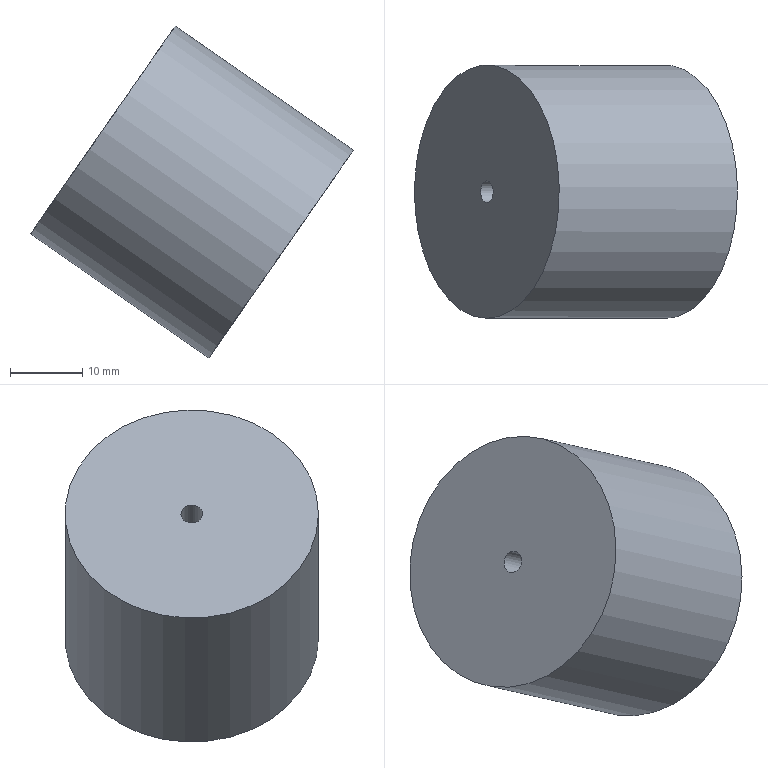Component | NX | SPROCKET_4 | 1 solid | 4 faces | box 44.62 x 35 x 45.87 mm | volume 28651 mm3 | cylinder 2 | plane 2 | commonest cylinder face diameters 35 x1 3 x1
STEP:
#1=CARTESIAN_POINT('',(0.,0.,0.));
#2=DIRECTION('',(0.,0.,1.));
#3=DIRECTION('',(1.,0.,0.));
#4=AXIS2_PLACEMENT_3D('',#1,#2,#3);
#5=CARTESIAN_POINT('',(273.351,21.806,77.155));
#6=VERTEX_POINT('',#5);
#7=CARTESIAN_POINT('',(275.944,4.905,80.88));
#8=DIRECTION('',(0.8207,-0.,-0.5713));
#9=DIRECTION('',(-0.1482,0.9658,-0.2129));
#10=AXIS2_PLACEMENT_3D('',#7,#8,#9);
#11=CIRCLE('',#10,17.5);
#12=CARTESIAN_POINT('',(275.944,4.905,80.88));
#13=DIRECTION('',(-0.8207,0.,0.5713));
#14=DIRECTION('',(0.1482,-0.9658,0.2129));
#15=AXIS2_PLACEMENT_3D('',#12,#13,#14);
#16=CYLINDRICAL_SURFACE('',#15,17.5);
#17=CARTESIAN_POINT('',(9.425,-0.));
#18=DIRECTION('',(-1.,0.));
#19=VECTOR('',#18,1.);
#20=LINE('',#17,#19);
#21=(GEOMETRIC_REPRESENTATION_CONTEXT(2)PARAMETRIC_REPRESENTATION_CONTEXT()REPRESENTATION_CONTEXT('',''));
#22=DEFINITIONAL_REPRESENTATION('',(#20),#21);
#23=PCURVE('',#16,#22);
#24=CARTESIAN_POINT('',(275.944,4.905,80.88));
#25=DIRECTION('',(0.8207,-0.,-0.5713));
#26=DIRECTION('',(-0.1482,0.9658,-0.2129));
#27=AXIS2_PLACEMENT_3D('',#24,#25,#26);
#28=PLANE('',#27);
#29=CARTESIAN_POINT('',(0.,0.));
#30=DIRECTION('',(1.,0.));
#31=AXIS2_PLACEMENT_2D('',#29,#30);
#32=CIRCLE('',#31,17.5);
#33=(GEOMETRIC_REPRESENTATION_CONTEXT(2)PARAMETRIC_REPRESENTATION_CONTEXT()REPRESENTATION_CONTEXT('',''));
#34=DEFINITIONAL_REPRESENTATION('',(#32),#33);
#35=PCURVE('',#28,#34);
#36=SURFACE_CURVE('',#11,(#23,#35),.PCURVE_S1.);
#37=EDGE_CURVE('',#6,#6,#36,.T.);
#38=ORIENTED_EDGE('',*,*,#37,.F.);
#39=CARTESIAN_POINT('',(248.729,21.806,94.295));
#40=VERTEX_POINT('',#39);
#41=CARTESIAN_POINT('',(273.351,21.806,77.155));
#42=CARTESIAN_POINT('',(248.729,21.806,94.295));
#43=B_SPLINE_CURVE_WITH_KNOTS('',1,(#41,#42),.UNSPECIFIED.,.F.,.F.,(2,2),(-0.,30.),.PIECEWISE_BEZIER_KNOTS.);
#44=CARTESIAN_POINT('',(9.425,0.));
#45=DIRECTION('',(0.,1.));
#46=VECTOR('',#45,1.);
#47=LINE('',#44,#46);
#48=(GEOMETRIC_REPRESENTATION_CONTEXT(2)PARAMETRIC_REPRESENTATION_CONTEXT()REPRESENTATION_CONTEXT('',''));
#49=DEFINITIONAL_REPRESENTATION('',(#47),#48);
#50=PCURVE('',#16,#49);
#51=CARTESIAN_POINT('',(3.142,0.));
#52=DIRECTION('',(0.,1.));
#53=VECTOR('',#52,1.);
#54=LINE('',#51,#53);
#55=(GEOMETRIC_REPRESENTATION_CONTEXT(2)PARAMETRIC_REPRESENTATION_CONTEXT()REPRESENTATION_CONTEXT('',''));
#56=DEFINITIONAL_REPRESENTATION('',(#54),#55);
#57=PCURVE('',#16,#56);
#58=SEAM_CURVE('',#43,(#50,#57),.PCURVE_S1.);
#59=EDGE_CURVE('',#6,#40,#58,.T.);
#60=ORIENTED_EDGE('',*,*,#59,.T.);
#61=CARTESIAN_POINT('',(251.322,4.905,98.02));
#62=DIRECTION('',(0.8207,-0.,-0.5713));
#63=DIRECTION('',(-0.1482,0.9658,-0.2129));
#64=AXIS2_PLACEMENT_3D('',#61,#62,#63);
#65=CIRCLE('',#64,17.5);
#66=CARTESIAN_POINT('',(9.425,30.));
#67=DIRECTION('',(-1.,0.));
#68=VECTOR('',#67,1.);
#69=LINE('',#66,#68);
#70=(GEOMETRIC_REPRESENTATION_CONTEXT(2)PARAMETRIC_REPRESENTATION_CONTEXT()REPRESENTATION_CONTEXT('',''));
#71=DEFINITIONAL_REPRESENTATION('',(#69),#70);
#72=PCURVE('',#16,#71);
#73=CARTESIAN_POINT('',(251.322,4.905,98.02));
#74=DIRECTION('',(0.8207,-0.,-0.5713));
#75=DIRECTION('',(-0.1482,0.9658,-0.2129));
#76=AXIS2_PLACEMENT_3D('',#73,#74,#75);
#77=PLANE('',#76);
#78=CARTESIAN_POINT('',(0.,0.));
#79=DIRECTION('',(1.,0.));
#80=AXIS2_PLACEMENT_2D('',#78,#79);
#81=CIRCLE('',#80,17.5);
#82=(GEOMETRIC_REPRESENTATION_CONTEXT(2)PARAMETRIC_REPRESENTATION_CONTEXT()REPRESENTATION_CONTEXT('',''));
#83=DEFINITIONAL_REPRESENTATION('',(#81),#82);
#84=PCURVE('',#77,#83);
#85=SURFACE_CURVE('',#65,(#72,#84),.PCURVE_S1.);
#86=EDGE_CURVE('',#40,#40,#85,.T.);
#87=ORIENTED_EDGE('',*,*,#86,.T.);
#88=ORIENTED_EDGE('',*,*,#59,.F.);
#89=EDGE_LOOP('',(#38,#60,#87,#88));
#90=FACE_BOUND('',#89,.T.);
#91=ADVANCED_FACE('',(#90),#16,.T.);
#92=CARTESIAN_POINT('',(276.166,3.456,81.2));
#93=VERTEX_POINT('',#92);
#94=CARTESIAN_POINT('',(275.944,4.905,80.88));
#95=DIRECTION('',(-0.8207,0.,0.5713));
#96=DIRECTION('',(0.1482,-0.9658,0.2129));
#97=AXIS2_PLACEMENT_3D('',#94,#95,#96);
#98=CIRCLE('',#97,1.5);
#99=CARTESIAN_POINT('',(-1.5,-0.));
#100=CARTESIAN_POINT('',(-1.5,2.598));
#101=CARTESIAN_POINT('',(0.75,1.299));
#102=CARTESIAN_POINT('',(3.,0.));
#103=CARTESIAN_POINT('',(0.75,-1.299));
#104=CARTESIAN_POINT('',(-1.5,-2.598));
#105=CARTESIAN_POINT('',(-1.5,-0.));
#106=(BOUNDED_CURVE()B_SPLINE_CURVE(2,(#99,#100,#101,#102,#103,#104,#105),.UNSPECIFIED.,.T.,.F.)B_SPLINE_CURVE_WITH_KNOTS((1,2,2,2,2,1),(-2.094,0.,2.094,4.189,6.283,8.378),.UNSPECIFIED.)CURVE()GEOMETRIC_REPRESENTATION_ITEM()RATIONAL_B_SPLINE_CURVE((1.,0.5,1.,0.5,1.,0.5,1.))REPRESENTATION_ITEM(''));
#107=(GEOMETRIC_REPRESENTATION_CONTEXT(2)PARAMETRIC_REPRESENTATION_CONTEXT()REPRESENTATION_CONTEXT('',''));
#108=DEFINITIONAL_REPRESENTATION('',(#106),#107);
#109=PCURVE('',#28,#108);
#110=CARTESIAN_POINT('',(275.944,4.905,80.88));
#111=DIRECTION('',(-0.8207,0.,0.5713));
#112=DIRECTION('',(0.1482,-0.9658,0.2129));
#113=AXIS2_PLACEMENT_3D('',#110,#111,#112);
#114=CYLINDRICAL_SURFACE('',#113,1.5);
#115=CARTESIAN_POINT('',(0.,0.));
#116=DIRECTION('',(1.,0.));
#117=VECTOR('',#116,1.);
#118=LINE('',#115,#117);
#119=(GEOMETRIC_REPRESENTATION_CONTEXT(2)PARAMETRIC_REPRESENTATION_CONTEXT()REPRESENTATION_CONTEXT('',''));
#120=DEFINITIONAL_REPRESENTATION('',(#118),#119);
#121=PCURVE('',#114,#120);
#122=SURFACE_CURVE('',#98,(#109,#121),.PCURVE_S1.);
#123=EDGE_CURVE('',#93,#93,#122,.T.);
#124=ORIENTED_EDGE('',*,*,#123,.T.);
#125=EDGE_LOOP('',(#124));
#126=FACE_BOUND('',#125,.T.);
#127=ORIENTED_EDGE('',*,*,#37,.T.);
#128=EDGE_LOOP('',(#127));
#129=FACE_BOUND('',#128,.T.);
#130=ADVANCED_FACE('',(#126,#129),#28,.T.);
#131=CARTESIAN_POINT('',(251.1,6.353,97.701));
#132=VERTEX_POINT('',#131);
#133=CARTESIAN_POINT('',(251.544,3.456,98.339));
#134=VERTEX_POINT('',#133);
#135=CARTESIAN_POINT('',(251.322,4.905,98.02));
#136=DIRECTION('',(0.8207,-0.,-0.5713));
#137=DIRECTION('',(-0.1482,0.9658,-0.2129));
#138=AXIS2_PLACEMENT_3D('',#135,#136,#137);
#139=CIRCLE('',#138,1.5);
#140=CARTESIAN_POINT('',(0.,0.));
#141=DIRECTION('',(1.,0.));
#142=AXIS2_PLACEMENT_2D('',#140,#141);
#143=CIRCLE('',#142,1.5);
#144=(GEOMETRIC_REPRESENTATION_CONTEXT(2)PARAMETRIC_REPRESENTATION_CONTEXT()REPRESENTATION_CONTEXT('',''));
#145=DEFINITIONAL_REPRESENTATION('',(#143),#144);
#146=PCURVE('',#77,#145);
#147=CARTESIAN_POINT('',(3.142,30.));
#148=DIRECTION('',(-1.,0.));
#149=VECTOR('',#148,1.);
#150=LINE('',#147,#149);
#151=(GEOMETRIC_REPRESENTATION_CONTEXT(2)PARAMETRIC_REPRESENTATION_CONTEXT()REPRESENTATION_CONTEXT('',''));
#152=DEFINITIONAL_REPRESENTATION('',(#150),#151);
#153=PCURVE('',#114,#152);
#154=SURFACE_CURVE('',#139,(#146,#153),.PCURVE_S1.);
#155=EDGE_CURVE('',#132,#134,#154,.T.);
#156=ORIENTED_EDGE('',*,*,#155,.T.);
#157=CARTESIAN_POINT('',(251.322,4.905,98.02));
#158=DIRECTION('',(0.8207,-0.,-0.5713));
#159=DIRECTION('',(-0.1482,0.9658,-0.2129));
#160=AXIS2_PLACEMENT_3D('',#157,#158,#159);
#161=CIRCLE('',#160,1.5);
#162=CARTESIAN_POINT('',(0.,0.));
#163=DIRECTION('',(1.,0.));
#164=AXIS2_PLACEMENT_2D('',#162,#163);
#165=CIRCLE('',#164,1.5);
#166=(GEOMETRIC_REPRESENTATION_CONTEXT(2)PARAMETRIC_REPRESENTATION_CONTEXT()REPRESENTATION_CONTEXT('',''));
#167=DEFINITIONAL_REPRESENTATION('',(#165),#166);
#168=PCURVE('',#77,#167);
#169=CARTESIAN_POINT('',(9.425,30.));
#170=DIRECTION('',(-1.,0.));
#171=VECTOR('',#170,1.);
#172=LINE('',#169,#171);
#173=(GEOMETRIC_REPRESENTATION_CONTEXT(2)PARAMETRIC_REPRESENTATION_CONTEXT()REPRESENTATION_CONTEXT('',''));
#174=DEFINITIONAL_REPRESENTATION('',(#172),#173);
#175=PCURVE('',#114,#174);
#176=SURFACE_CURVE('',#161,(#168,#175),.PCURVE_S1.);
#177=EDGE_CURVE('',#134,#132,#176,.T.);
#178=ORIENTED_EDGE('',*,*,#177,.T.);
#179=EDGE_LOOP('',(#156,#178));
#180=FACE_BOUND('',#179,.T.);
#181=ORIENTED_EDGE('',*,*,#86,.F.);
#182=EDGE_LOOP('',(#181));
#183=FACE_BOUND('',#182,.T.);
#184=ADVANCED_FACE('',(#180,#183),#77,.F.);
#185=ORIENTED_EDGE('',*,*,#123,.T.);
#186=CARTESIAN_POINT('',(276.166,3.456,81.2));
#187=CARTESIAN_POINT('',(251.544,3.456,98.339));
#188=B_SPLINE_CURVE_WITH_KNOTS('',1,(#186,#187),.UNSPECIFIED.,.F.,.F.,(2,2),(0.,30.),.PIECEWISE_BEZIER_KNOTS.);
#189=CARTESIAN_POINT('',(6.283,0.));
#190=DIRECTION('',(0.,1.));
#191=VECTOR('',#190,1.);
#192=LINE('',#189,#191);
#193=(GEOMETRIC_REPRESENTATION_CONTEXT(2)PARAMETRIC_REPRESENTATION_CONTEXT()REPRESENTATION_CONTEXT('',''));
#194=DEFINITIONAL_REPRESENTATION('',(#192),#193);
#195=PCURVE('',#114,#194);
#196=CARTESIAN_POINT('',(0.,0.));
#197=DIRECTION('',(0.,1.));
#198=VECTOR('',#197,1.);
#199=LINE('',#196,#198);
#200=(GEOMETRIC_REPRESENTATION_CONTEXT(2)PARAMETRIC_REPRESENTATION_CONTEXT()REPRESENTATION_CONTEXT('',''));
#201=DEFINITIONAL_REPRESENTATION('',(#199),#200);
#202=PCURVE('',#114,#201);
#203=SEAM_CURVE('',#188,(#195,#202),.PCURVE_S1.);
#204=EDGE_CURVE('',#93,#134,#203,.T.);
#205=ORIENTED_EDGE('',*,*,#204,.T.);
#206=ORIENTED_EDGE('',*,*,#177,.T.);
#207=ORIENTED_EDGE('',*,*,#155,.T.);
#208=ORIENTED_EDGE('',*,*,#204,.F.);
#209=EDGE_LOOP('',(#185,#205,#206,#207,#208));
#210=FACE_BOUND('',#209,.F.);
#211=ADVANCED_FACE('',(#210),#114,.F.);
#212=CLOSED_SHELL('',(#91,#130,#184,#211));
#213=MANIFOLD_SOLID_BREP('',#212);
#214=(LENGTH_UNIT()NAMED_UNIT(*)SI_UNIT(.MILLI.,.METRE.));
#215=UNCERTAINTY_MEASURE_WITH_UNIT(LENGTH_MEASURE(0.000005),#214,'','');
#216=(NAMED_UNIT(*)PLANE_ANGLE_UNIT()SI_UNIT($,.RADIAN.));
#217=(NAMED_UNIT(*)SI_UNIT($,.STERADIAN.)SOLID_ANGLE_UNIT());
#218=(GEOMETRIC_REPRESENTATION_CONTEXT(3)GLOBAL_UNCERTAINTY_ASSIGNED_CONTEXT((#215))GLOBAL_UNIT_ASSIGNED_CONTEXT((#214,#216,#217))REPRESENTATION_CONTEXT('',''));
#219=ADVANCED_BREP_SHAPE_REPRESENTATION('',(#4,#213),#218);